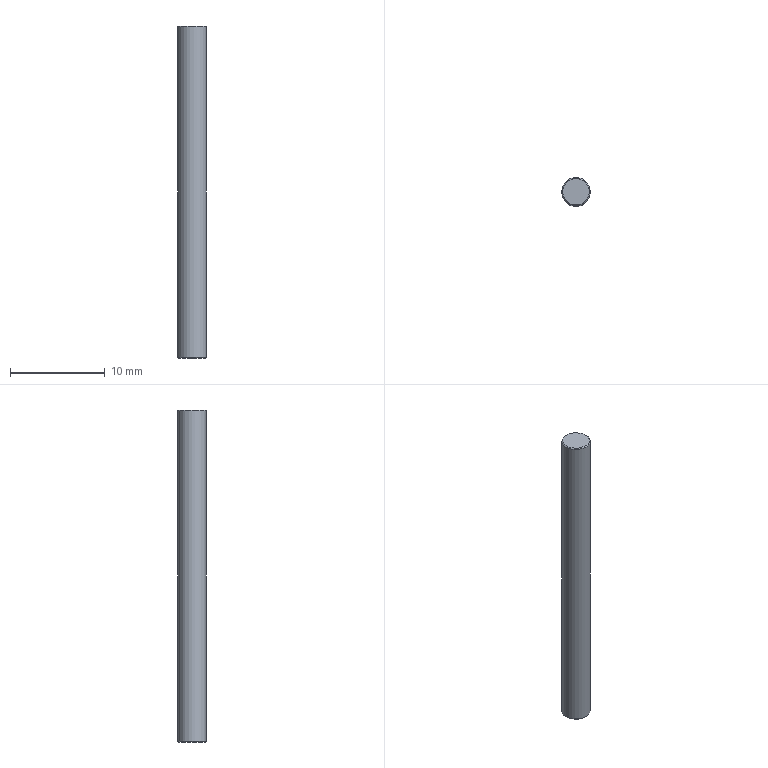Component | NX | STEPPER_SHAFT | 1 solid | 5 faces | box 3 x 3 x 35 mm | volume 247 mm3 | plane 2 | cone 2 | cylinder 1 | commonest cylinder face diameters 3 x1
STEP:
#1=CARTESIAN_POINT('',(0.,0.,0.));
#2=DIRECTION('',(0.,0.,1.));
#3=DIRECTION('',(1.,0.,0.));
#4=AXIS2_PLACEMENT_3D('',#1,#2,#3);
#5=CARTESIAN_POINT('',(1.5,-0.,6.));
#6=VERTEX_POINT('',#5);
#7=CARTESIAN_POINT('',(-0.,-0.,6.));
#8=DIRECTION('',(0.,0.,1.));
#9=DIRECTION('',(1.,0.,0.));
#10=AXIS2_PLACEMENT_3D('',#7,#8,#9);
#11=CIRCLE('',#10,1.5);
#12=CARTESIAN_POINT('',(-0.,-0.,40.9));
#13=DIRECTION('',(0.,0.,-1.));
#14=DIRECTION('',(-1.,0.,0.));
#15=AXIS2_PLACEMENT_3D('',#12,#13,#14);
#16=CYLINDRICAL_SURFACE('',#15,1.5);
#17=CARTESIAN_POINT('',(9.425,34.9));
#18=DIRECTION('',(-1.,0.));
#19=VECTOR('',#18,1.);
#20=LINE('',#17,#19);
#21=(GEOMETRIC_REPRESENTATION_CONTEXT(2)PARAMETRIC_REPRESENTATION_CONTEXT()REPRESENTATION_CONTEXT('',''));
#22=DEFINITIONAL_REPRESENTATION('',(#20),#21);
#23=PCURVE('',#16,#22);
#24=CARTESIAN_POINT('',(-0.,-0.,6.));
#25=DIRECTION('',(0.,0.,1.));
#26=DIRECTION('',(1.,0.,0.));
#27=AXIS2_PLACEMENT_3D('',#24,#25,#26);
#28=CONICAL_SURFACE('',#27,1.5,0.7854);
#29=CARTESIAN_POINT('',(0.,0.));
#30=DIRECTION('',(1.,0.));
#31=VECTOR('',#30,1.);
#32=LINE('',#29,#31);
#33=(GEOMETRIC_REPRESENTATION_CONTEXT(2)PARAMETRIC_REPRESENTATION_CONTEXT()REPRESENTATION_CONTEXT('',''));
#34=DEFINITIONAL_REPRESENTATION('',(#32),#33);
#35=PCURVE('',#28,#34);
#36=SURFACE_CURVE('',#11,(#23,#35),.PCURVE_S1.);
#37=EDGE_CURVE('',#6,#6,#36,.T.);
#38=ORIENTED_EDGE('',*,*,#37,.T.);
#39=CARTESIAN_POINT('',(1.5,-0.,40.8));
#40=VERTEX_POINT('',#39);
#41=CARTESIAN_POINT('',(1.5,-0.,40.8));
#42=CARTESIAN_POINT('',(1.5,-0.,6.));
#43=B_SPLINE_CURVE_WITH_KNOTS('',1,(#41,#42),.UNSPECIFIED.,.F.,.F.,(2,2),(0.1,34.9),.PIECEWISE_BEZIER_KNOTS.);
#44=CARTESIAN_POINT('',(3.142,0.));
#45=DIRECTION('',(0.,1.));
#46=VECTOR('',#45,1.);
#47=LINE('',#44,#46);
#48=(GEOMETRIC_REPRESENTATION_CONTEXT(2)PARAMETRIC_REPRESENTATION_CONTEXT()REPRESENTATION_CONTEXT('',''));
#49=DEFINITIONAL_REPRESENTATION('',(#47),#48);
#50=PCURVE('',#16,#49);
#51=CARTESIAN_POINT('',(9.425,0.));
#52=DIRECTION('',(0.,1.));
#53=VECTOR('',#52,1.);
#54=LINE('',#51,#53);
#55=(GEOMETRIC_REPRESENTATION_CONTEXT(2)PARAMETRIC_REPRESENTATION_CONTEXT()REPRESENTATION_CONTEXT('',''));
#56=DEFINITIONAL_REPRESENTATION('',(#54),#55);
#57=PCURVE('',#16,#56);
#58=SEAM_CURVE('',#43,(#50,#57),.PCURVE_S1.);
#59=EDGE_CURVE('',#40,#6,#58,.T.);
#60=ORIENTED_EDGE('',*,*,#59,.F.);
#61=CARTESIAN_POINT('',(-0.,-0.,40.8));
#62=DIRECTION('',(0.,0.,-1.));
#63=DIRECTION('',(1.,0.,0.));
#64=AXIS2_PLACEMENT_3D('',#61,#62,#63);
#65=CIRCLE('',#64,1.5);
#66=CARTESIAN_POINT('',(3.142,0.1));
#67=DIRECTION('',(1.,0.));
#68=VECTOR('',#67,1.);
#69=LINE('',#66,#68);
#70=(GEOMETRIC_REPRESENTATION_CONTEXT(2)PARAMETRIC_REPRESENTATION_CONTEXT()REPRESENTATION_CONTEXT('',''));
#71=DEFINITIONAL_REPRESENTATION('',(#69),#70);
#72=PCURVE('',#16,#71);
#73=CARTESIAN_POINT('',(-0.,-0.,40.9));
#74=DIRECTION('',(0.,0.,-1.));
#75=DIRECTION('',(-1.,0.,0.));
#76=AXIS2_PLACEMENT_3D('',#73,#74,#75);
#77=CONICAL_SURFACE('',#76,1.4,0.7854);
#78=CARTESIAN_POINT('',(3.142,0.1));
#79=DIRECTION('',(1.,0.));
#80=VECTOR('',#79,1.);
#81=LINE('',#78,#80);
#82=(GEOMETRIC_REPRESENTATION_CONTEXT(2)PARAMETRIC_REPRESENTATION_CONTEXT()REPRESENTATION_CONTEXT('',''));
#83=DEFINITIONAL_REPRESENTATION('',(#81),#82);
#84=PCURVE('',#77,#83);
#85=SURFACE_CURVE('',#65,(#72,#84),.PCURVE_S1.);
#86=EDGE_CURVE('',#40,#40,#85,.T.);
#87=ORIENTED_EDGE('',*,*,#86,.T.);
#88=ORIENTED_EDGE('',*,*,#59,.T.);
#89=EDGE_LOOP('',(#38,#60,#87,#88));
#90=FACE_BOUND('',#89,.T.);
#91=ADVANCED_FACE('',(#90),#16,.T.);
#92=CARTESIAN_POINT('',(1.4,-0.,40.9));
#93=VERTEX_POINT('',#92);
#94=CARTESIAN_POINT('',(-0.,-0.,40.9));
#95=DIRECTION('',(0.,0.,1.));
#96=DIRECTION('',(1.,0.,0.));
#97=AXIS2_PLACEMENT_3D('',#94,#95,#96);
#98=CIRCLE('',#97,1.4);
#99=CARTESIAN_POINT('',(-0.,-0.,40.9));
#100=DIRECTION('',(0.,0.,1.));
#101=DIRECTION('',(1.,0.,0.));
#102=AXIS2_PLACEMENT_3D('',#99,#100,#101);
#103=PLANE('',#102);
#104=CARTESIAN_POINT('',(0.,0.));
#105=DIRECTION('',(1.,0.));
#106=AXIS2_PLACEMENT_2D('',#104,#105);
#107=CIRCLE('',#106,1.4);
#108=(GEOMETRIC_REPRESENTATION_CONTEXT(2)PARAMETRIC_REPRESENTATION_CONTEXT()REPRESENTATION_CONTEXT('',''));
#109=DEFINITIONAL_REPRESENTATION('',(#107),#108);
#110=PCURVE('',#103,#109);
#111=CARTESIAN_POINT('',(9.425,0.));
#112=DIRECTION('',(-1.,0.));
#113=VECTOR('',#112,1.);
#114=LINE('',#111,#113);
#115=(GEOMETRIC_REPRESENTATION_CONTEXT(2)PARAMETRIC_REPRESENTATION_CONTEXT()REPRESENTATION_CONTEXT('',''));
#116=DEFINITIONAL_REPRESENTATION('',(#114),#115);
#117=PCURVE('',#77,#116);
#118=SURFACE_CURVE('',#98,(#110,#117),.PCURVE_S1.);
#119=EDGE_CURVE('',#93,#93,#118,.T.);
#120=ORIENTED_EDGE('',*,*,#119,.T.);
#121=EDGE_LOOP('',(#120));
#122=FACE_BOUND('',#121,.T.);
#123=ADVANCED_FACE('',(#122),#103,.T.);
#124=CARTESIAN_POINT('',(1.4,-0.,5.9));
#125=VERTEX_POINT('',#124);
#126=CARTESIAN_POINT('',(-0.,-0.,5.9));
#127=DIRECTION('',(0.,0.,-1.));
#128=DIRECTION('',(1.,0.,0.));
#129=AXIS2_PLACEMENT_3D('',#126,#127,#128);
#130=CIRCLE('',#129,1.4);
#131=CARTESIAN_POINT('',(-0.,-0.,5.9));
#132=DIRECTION('',(0.,0.,1.));
#133=DIRECTION('',(1.,0.,0.));
#134=AXIS2_PLACEMENT_3D('',#131,#132,#133);
#135=PLANE('',#134);
#136=CARTESIAN_POINT('',(1.4,0.));
#137=CARTESIAN_POINT('',(1.4,-2.425));
#138=CARTESIAN_POINT('',(-0.7,-1.212));
#139=CARTESIAN_POINT('',(-2.8,-0.));
#140=CARTESIAN_POINT('',(-0.7,1.212));
#141=CARTESIAN_POINT('',(1.4,2.425));
#142=CARTESIAN_POINT('',(1.4,0.));
#143=(BOUNDED_CURVE()B_SPLINE_CURVE(2,(#136,#137,#138,#139,#140,#141,#142),.UNSPECIFIED.,.T.,.F.)B_SPLINE_CURVE_WITH_KNOTS((1,2,2,2,2,1),(-2.094,0.,2.094,4.189,6.283,8.378),.UNSPECIFIED.)CURVE()GEOMETRIC_REPRESENTATION_ITEM()RATIONAL_B_SPLINE_CURVE((1.,0.5,1.,0.5,1.,0.5,1.))REPRESENTATION_ITEM(''));
#144=(GEOMETRIC_REPRESENTATION_CONTEXT(2)PARAMETRIC_REPRESENTATION_CONTEXT()REPRESENTATION_CONTEXT('',''));
#145=DEFINITIONAL_REPRESENTATION('',(#143),#144);
#146=PCURVE('',#135,#145);
#147=CARTESIAN_POINT('',(6.283,-0.1));
#148=DIRECTION('',(-1.,0.));
#149=VECTOR('',#148,1.);
#150=LINE('',#147,#149);
#151=(GEOMETRIC_REPRESENTATION_CONTEXT(2)PARAMETRIC_REPRESENTATION_CONTEXT()REPRESENTATION_CONTEXT('',''));
#152=DEFINITIONAL_REPRESENTATION('',(#150),#151);
#153=PCURVE('',#28,#152);
#154=SURFACE_CURVE('',#130,(#146,#153),.PCURVE_S1.);
#155=EDGE_CURVE('',#125,#125,#154,.T.);
#156=ORIENTED_EDGE('',*,*,#155,.T.);
#157=EDGE_LOOP('',(#156));
#158=FACE_BOUND('',#157,.T.);
#159=ADVANCED_FACE('',(#158),#135,.F.);
#160=ORIENTED_EDGE('',*,*,#155,.F.);
#161=CARTESIAN_POINT('',(1.4,-0.,5.9));
#162=CARTESIAN_POINT('',(1.5,-0.,6.));
#163=B_SPLINE_CURVE_WITH_KNOTS('',1,(#161,#162),.UNSPECIFIED.,.F.,.F.,(2,2),(-0.1414,0.),.PIECEWISE_BEZIER_KNOTS.);
#164=CARTESIAN_POINT('',(6.283,0.));
#165=DIRECTION('',(0.,1.));
#166=VECTOR('',#165,1.);
#167=LINE('',#164,#166);
#168=(GEOMETRIC_REPRESENTATION_CONTEXT(2)PARAMETRIC_REPRESENTATION_CONTEXT()REPRESENTATION_CONTEXT('',''));
#169=DEFINITIONAL_REPRESENTATION('',(#167),#168);
#170=PCURVE('',#28,#169);
#171=CARTESIAN_POINT('',(0.,0.));
#172=DIRECTION('',(0.,1.));
#173=VECTOR('',#172,1.);
#174=LINE('',#171,#173);
#175=(GEOMETRIC_REPRESENTATION_CONTEXT(2)PARAMETRIC_REPRESENTATION_CONTEXT()REPRESENTATION_CONTEXT('',''));
#176=DEFINITIONAL_REPRESENTATION('',(#174),#175);
#177=PCURVE('',#28,#176);
#178=SEAM_CURVE('',#163,(#170,#177),.PCURVE_S1.);
#179=EDGE_CURVE('',#125,#6,#178,.T.);
#180=ORIENTED_EDGE('',*,*,#179,.T.);
#181=ORIENTED_EDGE('',*,*,#37,.F.);
#182=ORIENTED_EDGE('',*,*,#179,.F.);
#183=EDGE_LOOP('',(#160,#180,#181,#182));
#184=FACE_BOUND('',#183,.T.);
#185=ADVANCED_FACE('',(#184),#28,.T.);
#186=ORIENTED_EDGE('',*,*,#86,.F.);
#187=CARTESIAN_POINT('',(1.4,-0.,40.9));
#188=CARTESIAN_POINT('',(1.5,-0.,40.8));
#189=B_SPLINE_CURVE_WITH_KNOTS('',1,(#187,#188),.UNSPECIFIED.,.F.,.F.,(2,2),(0.,0.1414),.PIECEWISE_BEZIER_KNOTS.);
#190=CARTESIAN_POINT('',(3.142,0.));
#191=DIRECTION('',(0.,1.));
#192=VECTOR('',#191,1.);
#193=LINE('',#190,#192);
#194=(GEOMETRIC_REPRESENTATION_CONTEXT(2)PARAMETRIC_REPRESENTATION_CONTEXT()REPRESENTATION_CONTEXT('',''));
#195=DEFINITIONAL_REPRESENTATION('',(#193),#194);
#196=PCURVE('',#77,#195);
#197=CARTESIAN_POINT('',(9.425,0.));
#198=DIRECTION('',(0.,1.));
#199=VECTOR('',#198,1.);
#200=LINE('',#197,#199);
#201=(GEOMETRIC_REPRESENTATION_CONTEXT(2)PARAMETRIC_REPRESENTATION_CONTEXT()REPRESENTATION_CONTEXT('',''));
#202=DEFINITIONAL_REPRESENTATION('',(#200),#201);
#203=PCURVE('',#77,#202);
#204=SEAM_CURVE('',#189,(#196,#203),.PCURVE_S1.);
#205=EDGE_CURVE('',#93,#40,#204,.T.);
#206=ORIENTED_EDGE('',*,*,#205,.F.);
#207=ORIENTED_EDGE('',*,*,#119,.F.);
#208=ORIENTED_EDGE('',*,*,#205,.T.);
#209=EDGE_LOOP('',(#186,#206,#207,#208));
#210=FACE_BOUND('',#209,.T.);
#211=ADVANCED_FACE('',(#210),#77,.T.);
#212=CLOSED_SHELL('',(#91,#123,#159,#185,#211));
#213=MANIFOLD_SOLID_BREP('',#212);
#214=(LENGTH_UNIT()NAMED_UNIT(*)SI_UNIT(.MILLI.,.METRE.));
#215=UNCERTAINTY_MEASURE_WITH_UNIT(LENGTH_MEASURE(0.00001),#214,'','');
#216=(NAMED_UNIT(*)PLANE_ANGLE_UNIT()SI_UNIT($,.RADIAN.));
#217=(NAMED_UNIT(*)SI_UNIT($,.STERADIAN.)SOLID_ANGLE_UNIT());
#218=(GEOMETRIC_REPRESENTATION_CONTEXT(3)GLOBAL_UNCERTAINTY_ASSIGNED_CONTEXT((#215))GLOBAL_UNIT_ASSIGNED_CONTEXT((#214,#216,#217))REPRESENTATION_CONTEXT('',''));
#219=ADVANCED_BREP_SHAPE_REPRESENTATION('',(#4,#213),#218);